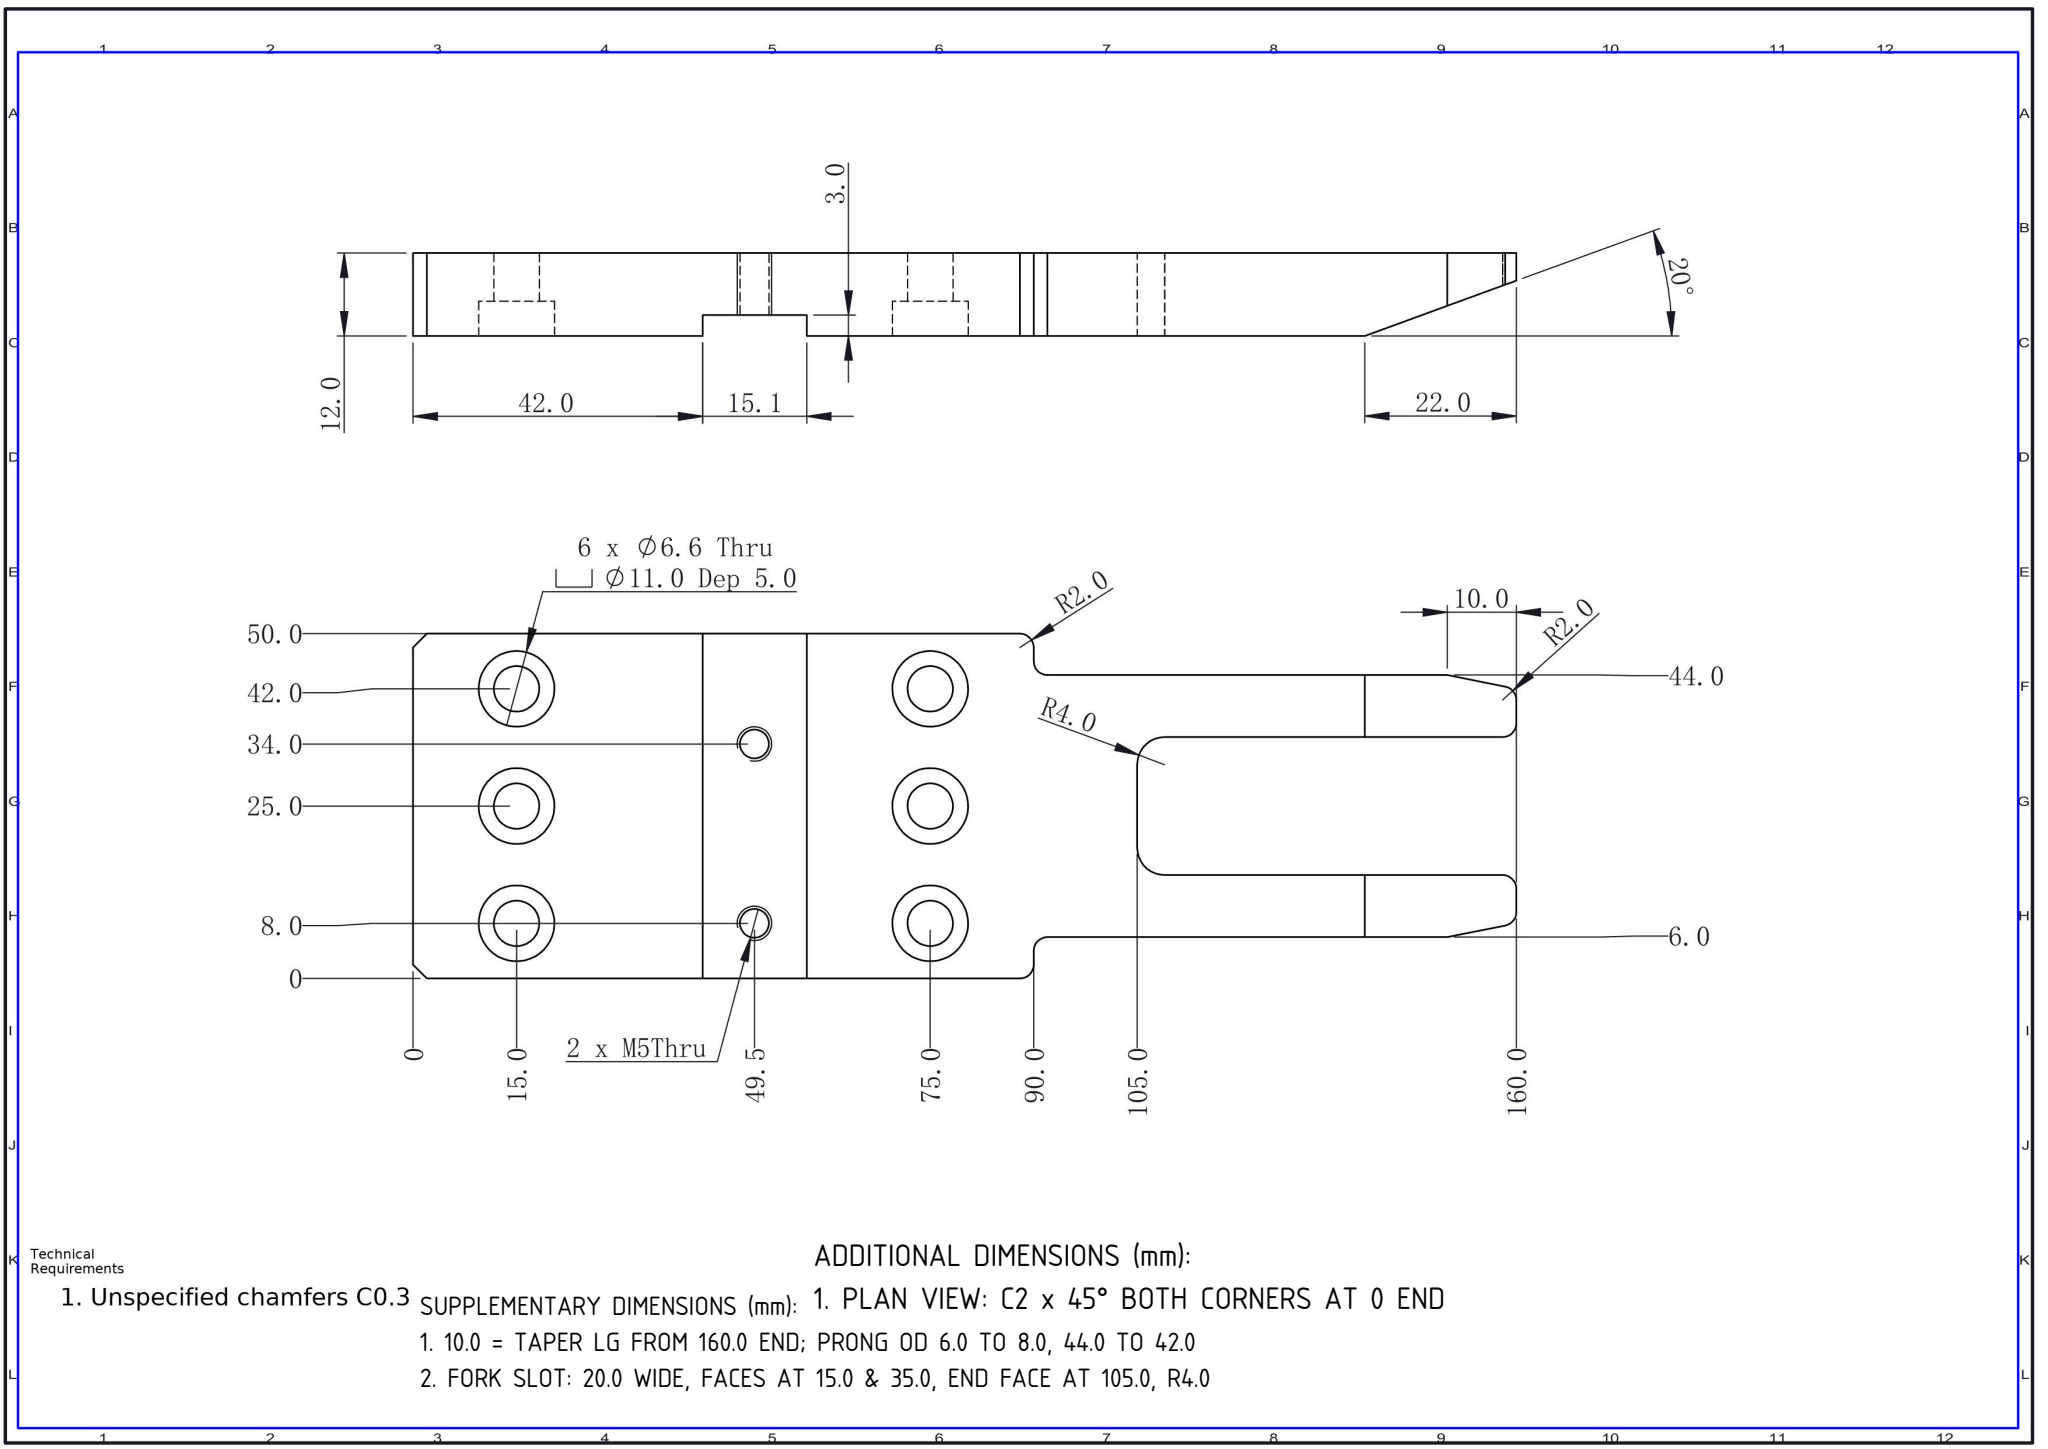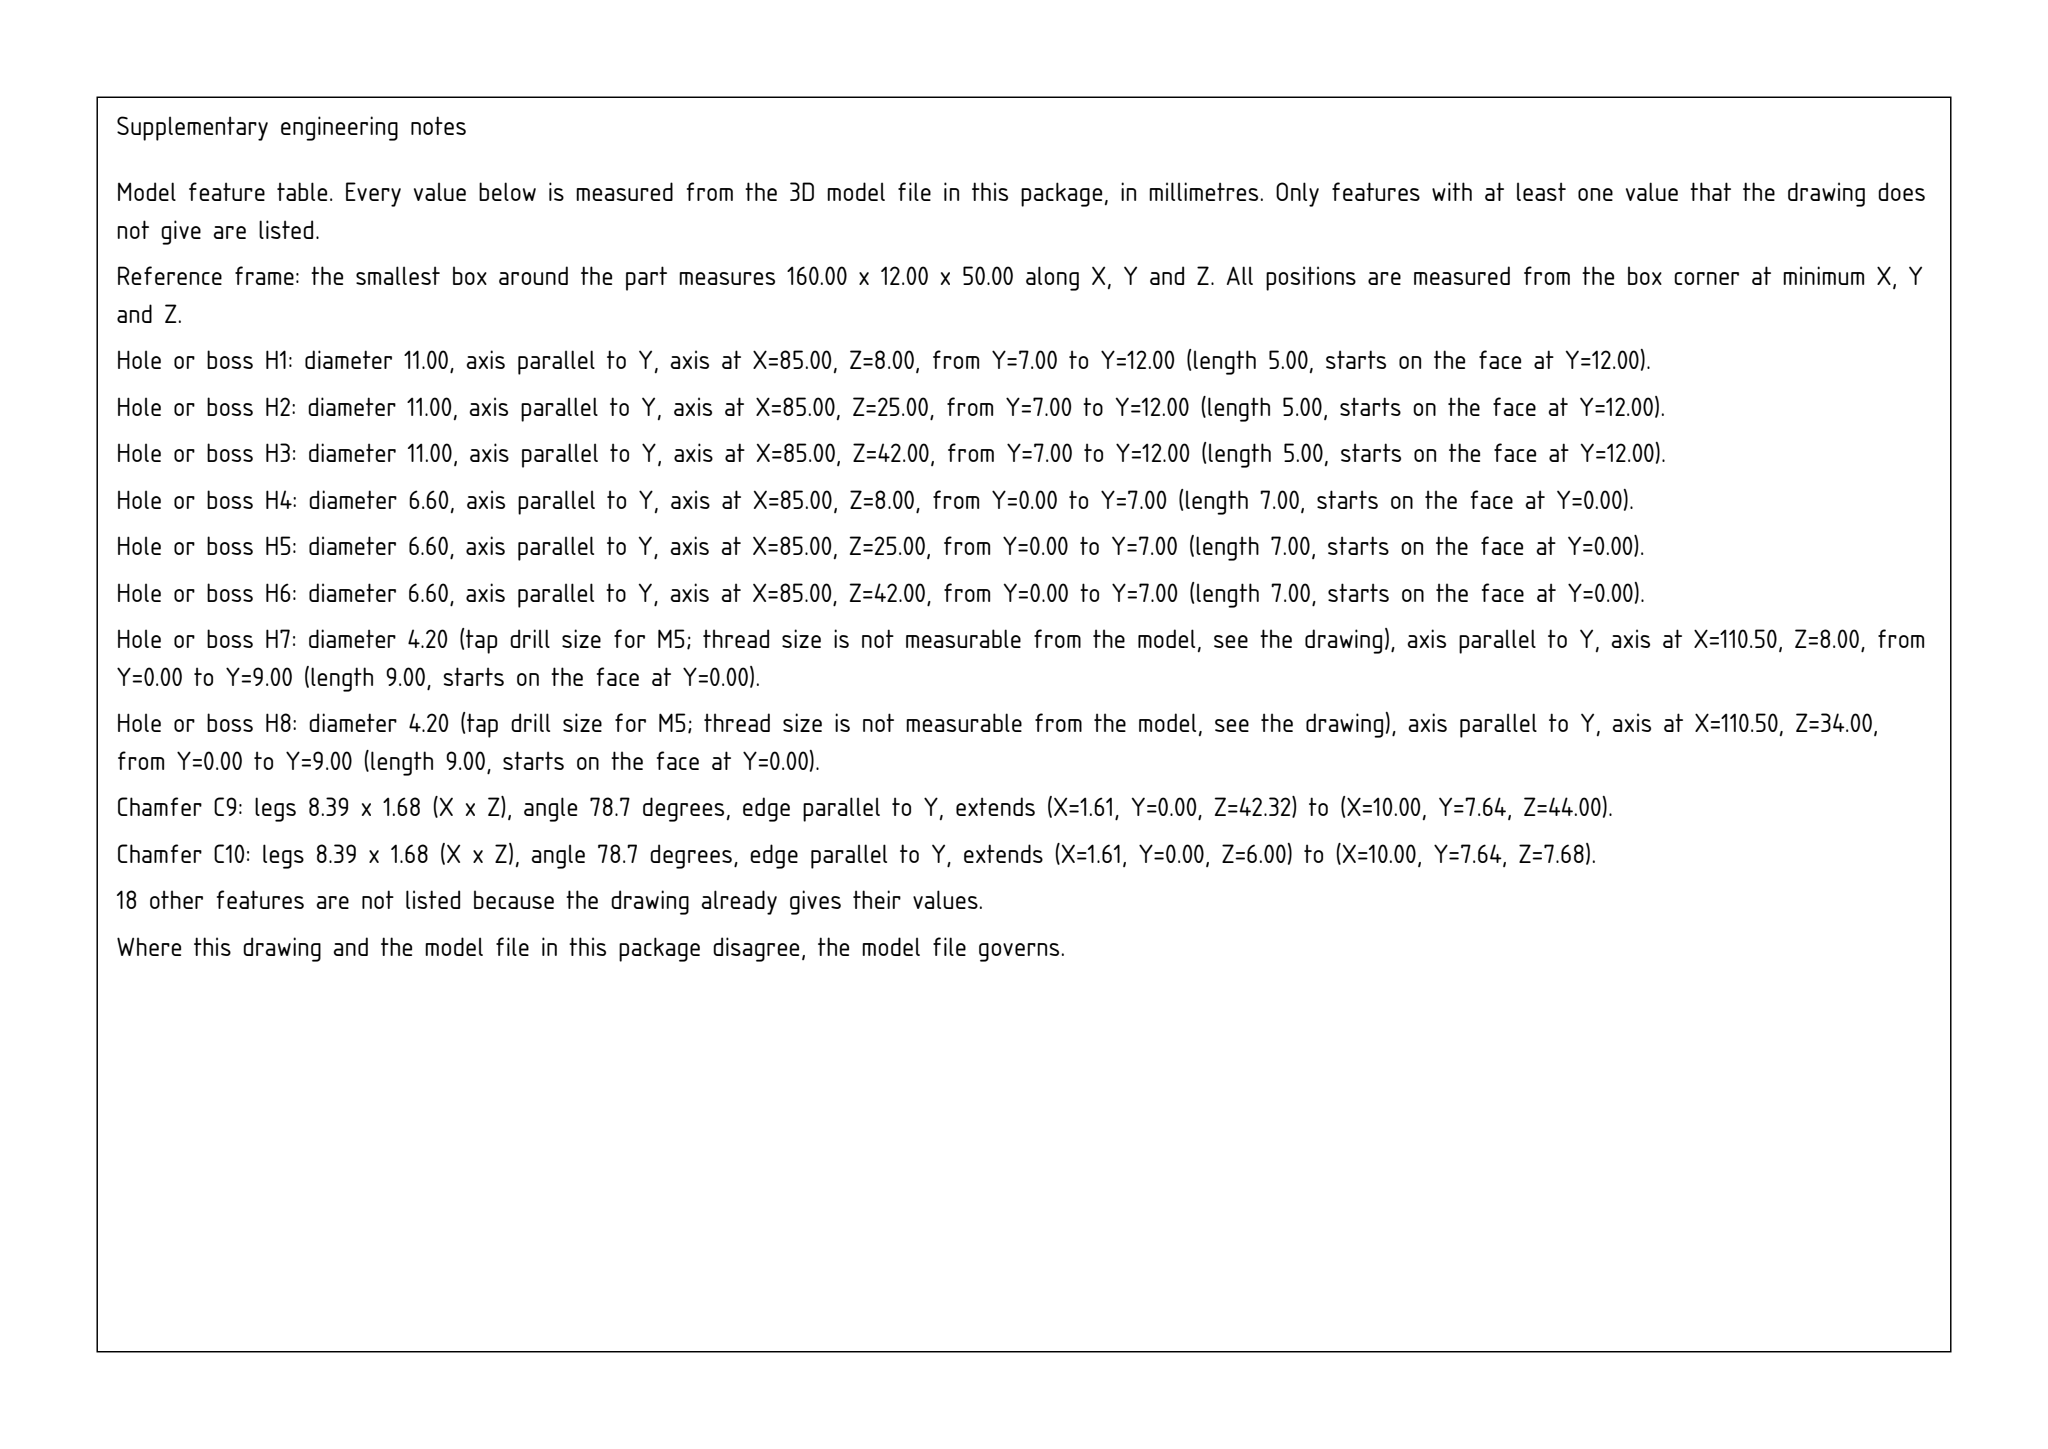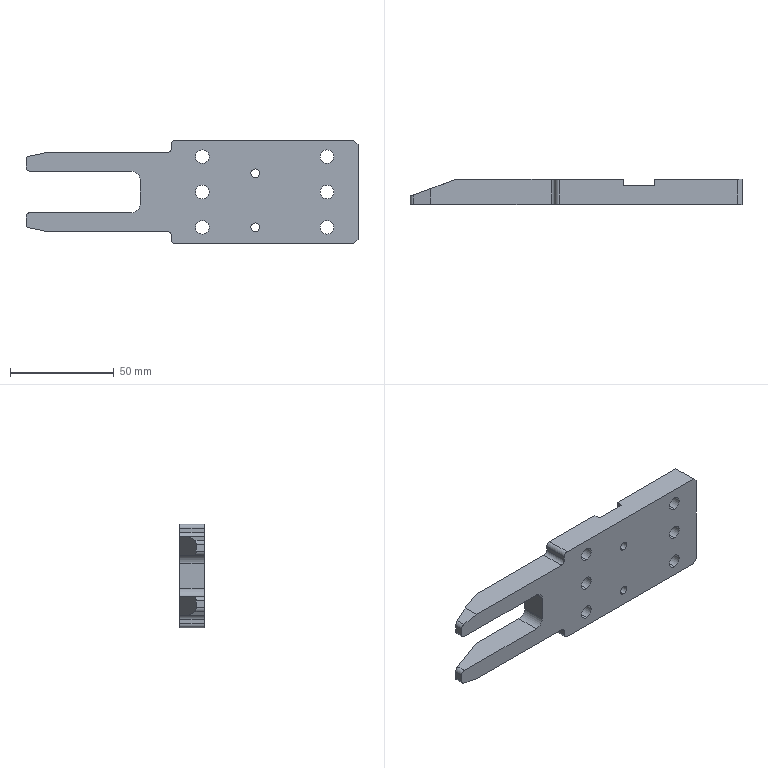Part | SolidWorks | mm | 1 solid | 68 faces | box 160 x 12 x 50 mm | volume 64254 mm3 | cylinder 38 | plane 30 | commonest cylinder face diameters 11 x12 6.6 x12 4 x8 4.2 x4 8 x2
build123d program:
from build123d import *

# Parameters (mm, degrees)
SKETCH1_W                                       = 160
SKETCH1_H                                       = 50
BOSS_EXTRUDE1_DEPTH                             = 6
M6_HEX_SOCKET_HEAD_CAP_SCREW_CBORE1_D           = 6.6
M6_HEX_SOCKET_HEAD_CAP_SCREW_CBORE1_CBORE_D     = 11
M6_HEX_SOCKET_HEAD_CAP_SCREW_CBORE1_CBORE_DEPTH = 5
SKETCH9_W                                       = 70
SKETCH9_H                                       = 6
CUT_EXTRUDE2_DEPTH                              = 85.67
FILLET1_R                                       = 2
CHAMFER1_SIZE                                   = 2
CHAMFER1_SIZE2                                  = 10
FILLET2_R                                       = 2
CHAMFER2_SIZE                                   = 2
CUT_EXTRUDE3_DEPTH                              = 92.499
SKETCH12_W                                      = 15.1
SKETCH12_H                                      = 50
CUT_EXTRUDE4_DEPTH                              = 3
M5_TAPPED_HOLE1_D                               = 4.2
SKETCH15_W                                      = 55
SKETCH15_H                                      = 20
CUT_EXTRUDE5_DEPTH                              = 85.67
FILLET3_R                                       = 4
FILLET4_R                                       = 2


with BuildPart() as part:
    # Sketch1 → Boss-Extrude1 (new, symmetric)
    with BuildSketch(Plane(origin=(0, 0, 0), x_dir=(1, 0, 0), z_dir=(0, 1, 0))):
        Rectangle(SKETCH1_W, SKETCH1_H)
    extrude(amount=BOSS_EXTRUDE1_DEPTH, both=True)

    # M6 Hex Socket Head Cap Screw CBORE1 (through all)
    with Locations(Plane(origin=(0, 6, 0), x_dir=(1, 0, 0), z_dir=(0, 1, 0))):
        with Locations((5, 17), (65, 17), (65, -17), (5, -17), (5, 0), (65, 0)):
            CounterBoreHole(M6_HEX_SOCKET_HEAD_CAP_SCREW_CBORE1_D / 2, M6_HEX_SOCKET_HEAD_CAP_SCREW_CBORE1_CBORE_D / 2, M6_HEX_SOCKET_HEAD_CAP_SCREW_CBORE1_CBORE_DEPTH)

    # Sketch9 → Cut-Extrude2 (cut, through all)
    with BuildSketch(Plane(origin=(0, 6, 0), x_dir=(1, 0, 0), z_dir=(0, 1, 0))):
        with Locations((-45, -22)):
            Rectangle(SKETCH9_W, SKETCH9_H)
        with Locations((-45, 22)):
            Rectangle(SKETCH9_W, SKETCH9_H)
    extrude(amount=-CUT_EXTRUDE2_DEPTH, mode=Mode.SUBTRACT)

    # Fillet1
    fillet1_edges = [part.edges().sort_by_distance(p)[0] for p in [
        (-10, 0, 19),
        (-10, 0, 25),
        (-10, 0, -25),
        (-10, 0, -19),
    ]]
    fillet(fillet1_edges, radius=FILLET1_R)

    # Chamfer1
    chamfer1_edges = [part.edges().sort_by_distance(p)[0] for p in [
        (-80, 0, 19),
        (-80, 0, -19),
    ]]
    chamfer1_side = [part.faces().sort_by_distance(p)[0] for p in [
        (-80, 0, 0),
    ]]
    chamfer(chamfer1_edges, length=CHAMFER1_SIZE, length2=CHAMFER1_SIZE2, reference=chamfer1_side[0])

    # Fillet2
    fillet2_edges = [part.edges().sort_by_distance(p)[0] for p in [
        (-80, 0, -17),
        (-80, 0, 17),
    ]]
    fillet(fillet2_edges, radius=FILLET2_R)

    # Chamfer2
    chamfer2_edges = [part.edges().sort_by_distance(p)[0] for p in [
        (80, 0, 25),
        (80, 0, -25),
    ]]
    chamfer(chamfer2_edges, length=CHAMFER2_SIZE)

    # Sketch10 → Cut-Extrude3 (cut, through all)
    with BuildSketch(Plane.XY.offset(19)):
        Polygon((-80, -2), (-58.02, 6), (-80, 6), align=None)
    extrude(amount=-CUT_EXTRUDE3_DEPTH, mode=Mode.SUBTRACT)

    # Sketch12 → Cut-Extrude4 (cut)
    with BuildSketch(Plane(origin=(0, 6, 0), x_dir=(1, 0, 0), z_dir=(0, 1, 0))):
        with Locations((30.45, 0)):
            Rectangle(SKETCH12_W, SKETCH12_H)
    extrude(amount=-CUT_EXTRUDE4_DEPTH, mode=Mode.SUBTRACT)

    # M5 Tapped Hole1 (through all)
    with Locations(Plane(origin=(0, 3, 0), x_dir=(1, 0, 0), z_dir=(0, 1, 0))):
        with Locations((30.5, -9), (30.5, 17)):
            Hole(M5_TAPPED_HOLE1_D / 2)

    # Sketch15 → Cut-Extrude5 (cut, through all)
    with BuildSketch(Plane(origin=(0, 6, 0), x_dir=(1, 0, 0), z_dir=(0, 1, 0))):
        with Locations((-52.5, 0)):
            Rectangle(SKETCH15_W, SKETCH15_H)
    extrude(amount=-CUT_EXTRUDE5_DEPTH, mode=Mode.SUBTRACT)

    # Fillet3
    fillet3_edges = [part.edges().sort_by_distance(p)[0] for p in [
        (-25, 0, 10),
        (-25, 0, -10),
    ]]
    fillet(fillet3_edges, radius=FILLET3_R)

    # Fillet4
    fillet4_edges = [part.edges().sort_by_distance(p)[0] for p in [
        (-80, -4, 10),
        (-80, -4, -10),
    ]]
    fillet(fillet4_edges, radius=FILLET4_R)


solid = part.part